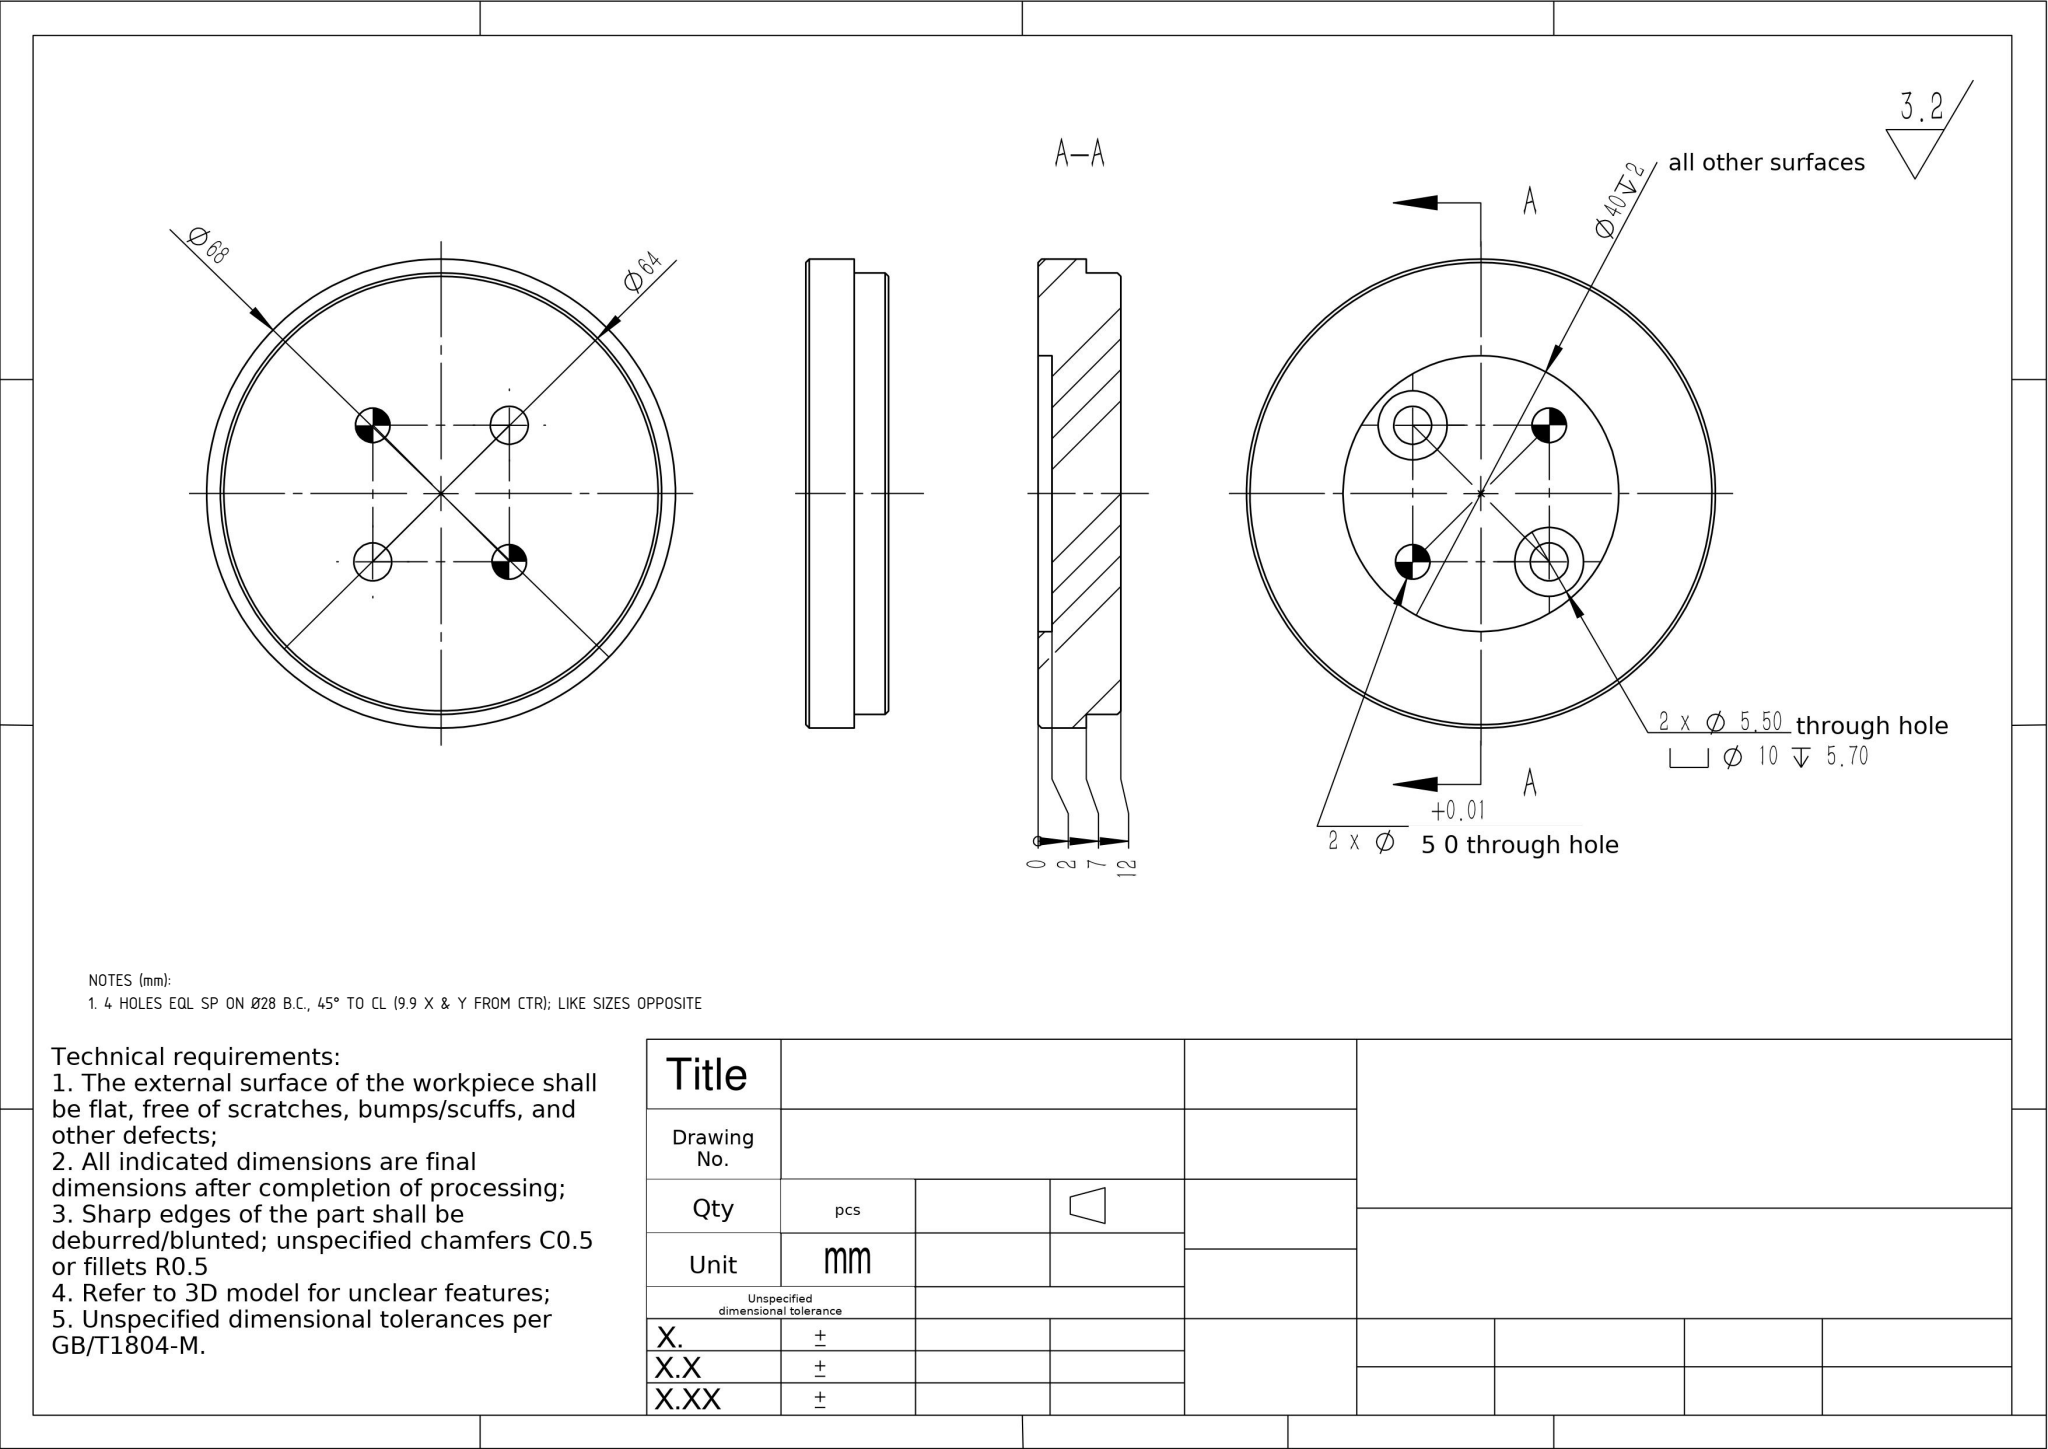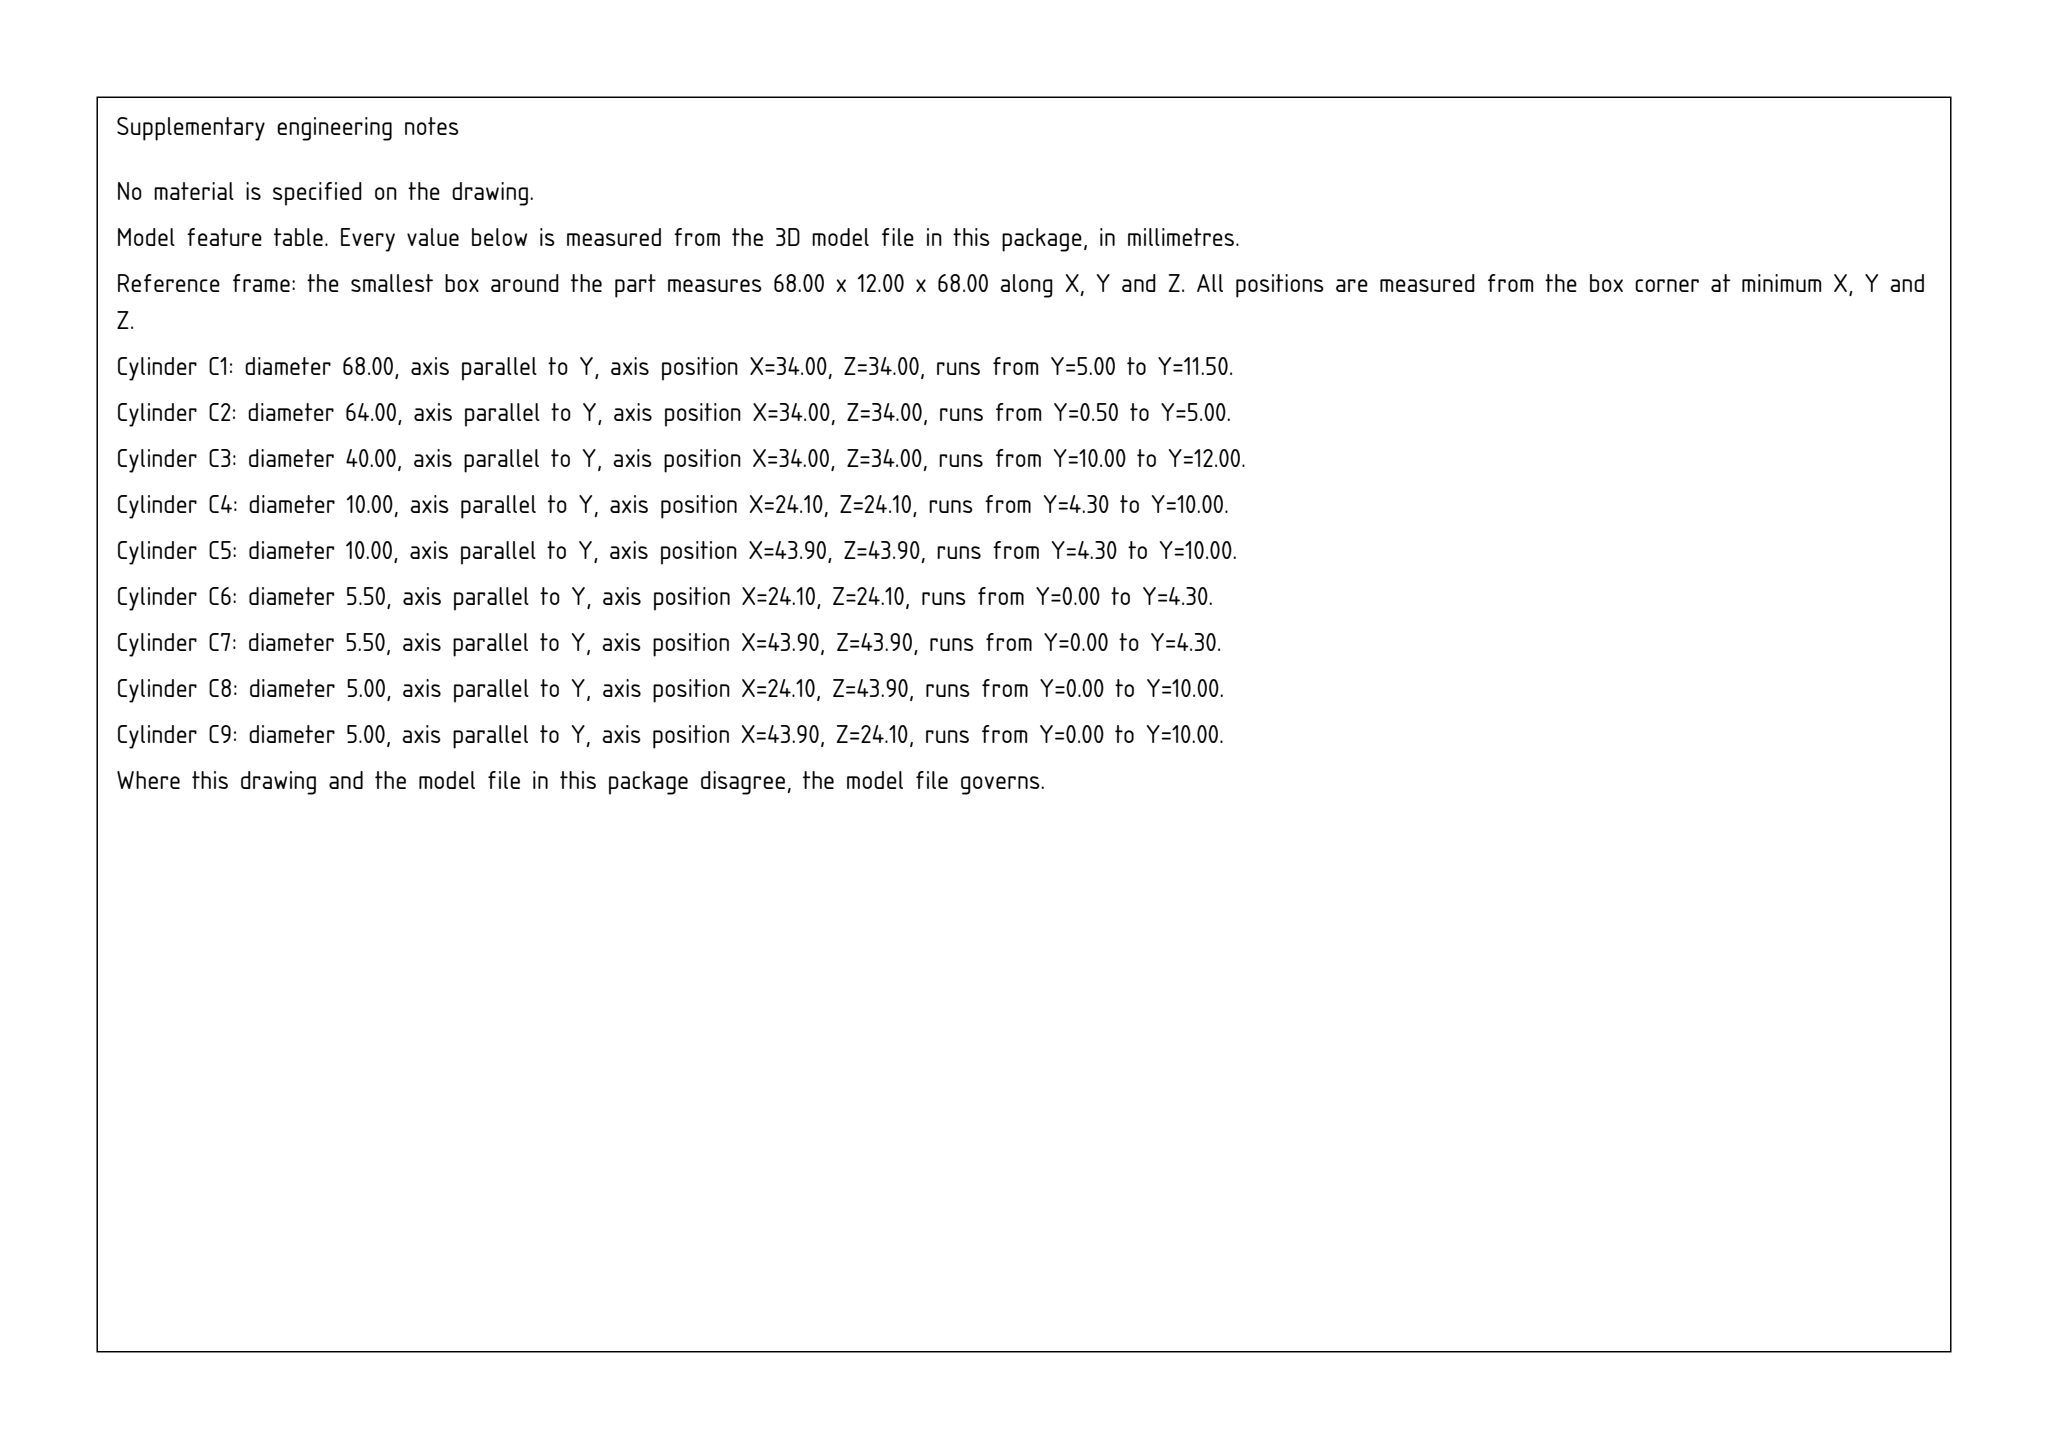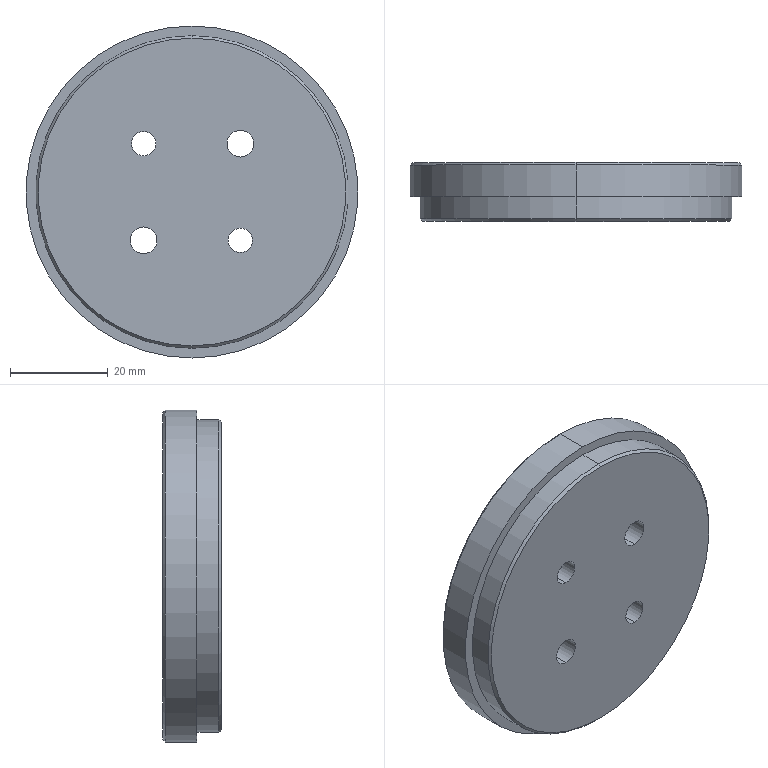Part | SolidWorks | mm | 1 solid | 28 faces | box 68 x 12 x 68 mm | volume 37449 mm3 | cylinder 18 | plane 6 | cone 4 | commonest cylinder face diameters 5 x4 10 x4 5.5 x4 40 x2 64 x2 68 x2
Drawing notes:
4 HOLES EQL SP ON Ø28 B.C., 45° TO CL (9.9 X & Y FROM CTR); LIKE SIZES OPPOSITE | from the solid: Ø5.5 at (24.1,24.1)&(43.9,43.9); Ø5.0 at (24.1,43.9)&(43.9,24.1); ctr 34,34; B.C.=2*sqrt(9.9²+9.9²)=28.0
build123d program:
from build123d import *

# Parameters (mm, degrees)
SKETCH1_R                                         = 34
BOSS_EXTRUDE1_DEPTH                               = 12
SKETCH5_R                                         = 34
SKETCH5_R_2                                       = 32
CUT_EXTRUDE2_DEPTH                                = 5
SKETCH9_R                                         = 20
CUT_EXTRUDE3_DEPTH                                = 2
HOLE_SIZE_ACCORDING_TO_HEXAGON_SOCKET_D           = 5.5
HOLE_SIZE_ACCORDING_TO_HEXAGON_SOCKET_CBORE_D     = 10
HOLE_SIZE_ACCORDING_TO_HEXAGON_SOCKET_CBORE_DEPTH = 5.7
SIZE_MM_DOWEL_PIN_HOLE_2_D                        = 5
CHAMFER1_SIZE                                     = 0.5


with BuildPart() as part:
    # Sketch1 → Boss-Extrude1 (new body)
    with BuildSketch(Plane(origin=(0, 0, 0), x_dir=(1, 0, 0), z_dir=(0, 1, 0))):
        with Locations(Location((0, 0, 0), (0, 0, 270))):
            Circle(SKETCH1_R)
    extrude(amount=BOSS_EXTRUDE1_DEPTH)

    # Sketch5 → Cut-Extrude2 (cut)
    with BuildSketch(Plane.XZ):
        with Locations(Location((0, 0, 0), (0, 0, 270))):
            Circle(SKETCH5_R)
        with Locations(Location((0, 0, 0), (0, 0, 270))):
            Circle(SKETCH5_R_2, mode=Mode.SUBTRACT)
    extrude(amount=-CUT_EXTRUDE2_DEPTH, mode=Mode.SUBTRACT)

    # Sketch9 → Cut-Extrude3 (cut)
    with BuildSketch(Plane(origin=(0, 12, 0), x_dir=(1, 0, 0), z_dir=(0, 1, 0))):
        with Locations(Location((0, 0, 0), (0, 0, 270))):
            Circle(SKETCH9_R)
    extrude(amount=-CUT_EXTRUDE3_DEPTH, mode=Mode.SUBTRACT)

    # Hole Size _ according to_ Hexagon Socket (through all)
    with Locations(Plane(origin=(-9.899, 10, -9.899), x_dir=(0, 0, 1), z_dir=(0, 1, 0))):
        with Locations((0, 0), (19.799, 19.799)):
            CounterBoreHole(HOLE_SIZE_ACCORDING_TO_HEXAGON_SOCKET_D / 2, HOLE_SIZE_ACCORDING_TO_HEXAGON_SOCKET_CBORE_D / 2, HOLE_SIZE_ACCORDING_TO_HEXAGON_SOCKET_CBORE_DEPTH)

    # Size mm Dowel Pin Hole 2 (through all)
    with Locations(Plane(origin=(-9.899, 10, 9.899), x_dir=(0, 0, 1), z_dir=(0, 1, 0))):
        with Locations((0, 0), (-19.799, 19.799)):
            Hole(SIZE_MM_DOWEL_PIN_HOLE_2_D / 2)

    # Chamfer1
    chamfer1_edges = [part.edges().sort_by_distance(p)[0] for p in [
        (0, 12, -34),
        (0, 0, 32),
    ]]
    chamfer(chamfer1_edges, length=CHAMFER1_SIZE)


solid = part.part
STEP:
#1=CARTESIAN_POINT('',(0.,12.,33.5));
#2=VERTEX_POINT('',#1);
#3=CARTESIAN_POINT('',(0.,12.,-33.5));
#4=VERTEX_POINT('',#3);
#5=CARTESIAN_POINT('',(0.,12.,0.));
#6=DIRECTION('',(0.,1.,0.));
#7=DIRECTION('',(0.,0.,1.));
#8=AXIS2_PLACEMENT_3D('',#5,#6,#7);
#9=CIRCLE('',#8,33.5);
#10=EDGE_CURVE('',#2,#4,#9,.T.);
#11=ORIENTED_EDGE('',*,*,#10,.F.);
#12=CARTESIAN_POINT('',(0.,11.5,34.));
#13=VERTEX_POINT('',#12);
#14=CARTESIAN_POINT('',(0.,12.,33.5));
#15=DIRECTION('',(0.,-0.7071,0.7071));
#16=VECTOR('',#15,1000.);
#17=LINE('',#14,#16);
#18=EDGE_CURVE('',#2,#13,#17,.T.);
#19=ORIENTED_EDGE('',*,*,#18,.T.);
#20=CARTESIAN_POINT('',(0.,11.5,-34.));
#21=VERTEX_POINT('',#20);
#22=CARTESIAN_POINT('',(0.,11.5,0.));
#23=DIRECTION('',(0.,-1.,0.));
#24=DIRECTION('',(0.,0.,1.));
#25=AXIS2_PLACEMENT_3D('',#22,#23,#24);
#26=CIRCLE('',#25,34.);
#27=EDGE_CURVE('',#21,#13,#26,.T.);
#28=ORIENTED_EDGE('',*,*,#27,.F.);
#29=CARTESIAN_POINT('',(0.,12.,-33.5));
#30=DIRECTION('',(0.,-0.7071,-0.7071));
#31=VECTOR('',#30,1000.);
#32=LINE('',#29,#31);
#33=EDGE_CURVE('',#4,#21,#32,.T.);
#34=ORIENTED_EDGE('',*,*,#33,.F.);
#35=EDGE_LOOP('',(#11,#19,#28,#34));
#36=FACE_OUTER_BOUND('',#35,.T.);
#37=CARTESIAN_POINT('',(0.,12.,0.));
#38=DIRECTION('',(0.,-1.,0.));
#39=DIRECTION('',(0.,0.,-1.));
#40=AXIS2_PLACEMENT_3D('',#37,#38,#39);
#41=CONICAL_SURFACE('',#40,33.5,0.7854);
#42=ADVANCED_FACE('',(#36),#41,.T.);
#43=CARTESIAN_POINT('',(0.,0.,-31.5));
#44=VERTEX_POINT('',#43);
#45=CARTESIAN_POINT('',(0.,0.,31.5));
#46=VERTEX_POINT('',#45);
#47=CARTESIAN_POINT('',(0.,0.,0.));
#48=DIRECTION('',(0.,-1.,0.));
#49=DIRECTION('',(0.,0.,1.));
#50=AXIS2_PLACEMENT_3D('',#47,#48,#49);
#51=CIRCLE('',#50,31.5);
#52=EDGE_CURVE('',#44,#46,#51,.T.);
#53=ORIENTED_EDGE('',*,*,#52,.F.);
#54=CARTESIAN_POINT('',(0.,0.5,-32.));
#55=VERTEX_POINT('',#54);
#56=CARTESIAN_POINT('',(0.,0.,-31.5));
#57=DIRECTION('',(0.,0.7071,-0.7071));
#58=VECTOR('',#57,1000.);
#59=LINE('',#56,#58);
#60=EDGE_CURVE('',#44,#55,#59,.T.);
#61=ORIENTED_EDGE('',*,*,#60,.T.);
#62=CARTESIAN_POINT('',(0.,0.5,32.));
#63=VERTEX_POINT('',#62);
#64=CARTESIAN_POINT('',(0.,0.5,0.));
#65=DIRECTION('',(0.,1.,0.));
#66=DIRECTION('',(0.,0.,1.));
#67=AXIS2_PLACEMENT_3D('',#64,#65,#66);
#68=CIRCLE('',#67,32.);
#69=EDGE_CURVE('',#63,#55,#68,.T.);
#70=ORIENTED_EDGE('',*,*,#69,.F.);
#71=CARTESIAN_POINT('',(0.,0.,31.5));
#72=DIRECTION('',(0.,0.7071,0.7071));
#73=VECTOR('',#72,1000.);
#74=LINE('',#71,#73);
#75=EDGE_CURVE('',#46,#63,#74,.T.);
#76=ORIENTED_EDGE('',*,*,#75,.F.);
#77=EDGE_LOOP('',(#53,#61,#70,#76));
#78=FACE_OUTER_BOUND('',#77,.T.);
#79=CARTESIAN_POINT('',(0.,0.,0.));
#80=DIRECTION('',(0.,1.,0.));
#81=DIRECTION('',(0.,0.,1.));
#82=AXIS2_PLACEMENT_3D('',#79,#80,#81);
#83=CONICAL_SURFACE('',#82,31.5,0.7854);
#84=ADVANCED_FACE('',(#78),#83,.T.);
#85=CARTESIAN_POINT('',(-9.899,0.,7.399));
#86=VERTEX_POINT('',#85);
#87=CARTESIAN_POINT('',(-9.899,0.,12.399));
#88=VERTEX_POINT('',#87);
#89=CARTESIAN_POINT('',(-9.899,0.,9.899));
#90=DIRECTION('',(0.,1.,0.));
#91=DIRECTION('',(0.,0.,1.));
#92=AXIS2_PLACEMENT_3D('',#89,#90,#91);
#93=CIRCLE('',#92,2.5);
#94=EDGE_CURVE('',#86,#88,#93,.T.);
#95=ORIENTED_EDGE('',*,*,#94,.F.);
#96=CARTESIAN_POINT('',(-9.899,10.,7.399));
#97=VERTEX_POINT('',#96);
#98=CARTESIAN_POINT('',(-9.899,10.,7.399));
#99=DIRECTION('',(0.,1.,0.));
#100=VECTOR('',#99,1000.);
#101=LINE('',#98,#100);
#102=EDGE_CURVE('',#86,#97,#101,.T.);
#103=ORIENTED_EDGE('',*,*,#102,.T.);
#104=CARTESIAN_POINT('',(-9.899,10.,12.399));
#105=VERTEX_POINT('',#104);
#106=CARTESIAN_POINT('',(-9.899,10.,9.899));
#107=DIRECTION('',(0.,1.,0.));
#108=DIRECTION('',(0.,0.,1.));
#109=AXIS2_PLACEMENT_3D('',#106,#107,#108);
#110=CIRCLE('',#109,2.5);
#111=EDGE_CURVE('',#97,#105,#110,.T.);
#112=ORIENTED_EDGE('',*,*,#111,.T.);
#113=CARTESIAN_POINT('',(-9.899,10.,12.399));
#114=DIRECTION('',(0.,1.,0.));
#115=VECTOR('',#114,1000.);
#116=LINE('',#113,#115);
#117=EDGE_CURVE('',#88,#105,#116,.T.);
#118=ORIENTED_EDGE('',*,*,#117,.F.);
#119=EDGE_LOOP('',(#95,#103,#112,#118));
#120=FACE_OUTER_BOUND('',#119,.T.);
#121=CARTESIAN_POINT('',(-9.899,10.,9.899));
#122=DIRECTION('',(0.,1.,0.));
#123=DIRECTION('',(0.,0.,1.));
#124=AXIS2_PLACEMENT_3D('',#121,#122,#123);
#125=CYLINDRICAL_SURFACE('',#124,2.5);
#126=ADVANCED_FACE('',(#120),#125,.F.);
#127=CARTESIAN_POINT('',(9.899,0.,-12.399));
#128=VERTEX_POINT('',#127);
#129=CARTESIAN_POINT('',(9.899,0.,-7.399));
#130=VERTEX_POINT('',#129);
#131=CARTESIAN_POINT('',(9.899,0.,-9.899));
#132=DIRECTION('',(0.,1.,0.));
#133=DIRECTION('',(0.,0.,1.));
#134=AXIS2_PLACEMENT_3D('',#131,#132,#133);
#135=CIRCLE('',#134,2.5);
#136=EDGE_CURVE('',#128,#130,#135,.T.);
#137=ORIENTED_EDGE('',*,*,#136,.F.);
#138=CARTESIAN_POINT('',(9.899,10.,-12.399));
#139=VERTEX_POINT('',#138);
#140=CARTESIAN_POINT('',(9.899,10.,-12.399));
#141=DIRECTION('',(0.,1.,0.));
#142=VECTOR('',#141,1000.);
#143=LINE('',#140,#142);
#144=EDGE_CURVE('',#128,#139,#143,.T.);
#145=ORIENTED_EDGE('',*,*,#144,.T.);
#146=CARTESIAN_POINT('',(9.899,10.,-7.399));
#147=VERTEX_POINT('',#146);
#148=CARTESIAN_POINT('',(9.899,10.,-9.899));
#149=DIRECTION('',(0.,1.,0.));
#150=DIRECTION('',(0.,0.,1.));
#151=AXIS2_PLACEMENT_3D('',#148,#149,#150);
#152=CIRCLE('',#151,2.5);
#153=EDGE_CURVE('',#139,#147,#152,.T.);
#154=ORIENTED_EDGE('',*,*,#153,.T.);
#155=CARTESIAN_POINT('',(9.899,10.,-7.399));
#156=DIRECTION('',(0.,1.,0.));
#157=VECTOR('',#156,1000.);
#158=LINE('',#155,#157);
#159=EDGE_CURVE('',#130,#147,#158,.T.);
#160=ORIENTED_EDGE('',*,*,#159,.F.);
#161=EDGE_LOOP('',(#137,#145,#154,#160));
#162=FACE_OUTER_BOUND('',#161,.T.);
#163=CARTESIAN_POINT('',(9.899,10.,-9.899));
#164=DIRECTION('',(0.,1.,0.));
#165=DIRECTION('',(0.,0.,1.));
#166=AXIS2_PLACEMENT_3D('',#163,#164,#165);
#167=CYLINDRICAL_SURFACE('',#166,2.5);
#168=ADVANCED_FACE('',(#162),#167,.F.);
#169=CARTESIAN_POINT('',(-9.899,4.3,-14.899));
#170=VERTEX_POINT('',#169);
#171=CARTESIAN_POINT('',(-9.899,4.3,-4.899));
#172=VERTEX_POINT('',#171);
#173=CARTESIAN_POINT('',(-9.899,4.3,-9.899));
#174=DIRECTION('',(0.,1.,0.));
#175=DIRECTION('',(0.,0.,1.));
#176=AXIS2_PLACEMENT_3D('',#173,#174,#175);
#177=CIRCLE('',#176,5.);
#178=EDGE_CURVE('',#170,#172,#177,.T.);
#179=ORIENTED_EDGE('',*,*,#178,.F.);
#180=CARTESIAN_POINT('',(-9.899,10.,-14.899));
#181=VERTEX_POINT('',#180);
#182=CARTESIAN_POINT('',(-9.899,10.,-14.899));
#183=DIRECTION('',(0.,1.,0.));
#184=VECTOR('',#183,1000.);
#185=LINE('',#182,#184);
#186=EDGE_CURVE('',#170,#181,#185,.T.);
#187=ORIENTED_EDGE('',*,*,#186,.T.);
#188=CARTESIAN_POINT('',(-9.899,10.,-4.899));
#189=VERTEX_POINT('',#188);
#190=CARTESIAN_POINT('',(-9.899,10.,-9.899));
#191=DIRECTION('',(0.,1.,0.));
#192=DIRECTION('',(0.,0.,1.));
#193=AXIS2_PLACEMENT_3D('',#190,#191,#192);
#194=CIRCLE('',#193,5.);
#195=EDGE_CURVE('',#181,#189,#194,.T.);
#196=ORIENTED_EDGE('',*,*,#195,.T.);
#197=CARTESIAN_POINT('',(-9.899,10.,-4.899));
#198=DIRECTION('',(0.,1.,0.));
#199=VECTOR('',#198,1000.);
#200=LINE('',#197,#199);
#201=EDGE_CURVE('',#172,#189,#200,.T.);
#202=ORIENTED_EDGE('',*,*,#201,.F.);
#203=EDGE_LOOP('',(#179,#187,#196,#202));
#204=FACE_OUTER_BOUND('',#203,.T.);
#205=CARTESIAN_POINT('',(-9.899,10.,-9.899));
#206=DIRECTION('',(0.,1.,0.));
#207=DIRECTION('',(0.,0.,1.));
#208=AXIS2_PLACEMENT_3D('',#205,#206,#207);
#209=CYLINDRICAL_SURFACE('',#208,5.);
#210=ADVANCED_FACE('',(#204),#209,.F.);
#211=CARTESIAN_POINT('',(-9.899,0.,-12.649));
#212=VERTEX_POINT('',#211);
#213=CARTESIAN_POINT('',(-9.899,0.,-7.149));
#214=VERTEX_POINT('',#213);
#215=CARTESIAN_POINT('',(-9.899,0.,-9.899));
#216=DIRECTION('',(0.,1.,0.));
#217=DIRECTION('',(0.,0.,1.));
#218=AXIS2_PLACEMENT_3D('',#215,#216,#217);
#219=CIRCLE('',#218,2.75);
#220=EDGE_CURVE('',#212,#214,#219,.T.);
#221=ORIENTED_EDGE('',*,*,#220,.F.);
#222=CARTESIAN_POINT('',(-9.899,4.3,-12.649));
#223=VERTEX_POINT('',#222);
#224=CARTESIAN_POINT('',(-9.899,10.,-12.649));
#225=DIRECTION('',(0.,1.,0.));
#226=VECTOR('',#225,1000.);
#227=LINE('',#224,#226);
#228=EDGE_CURVE('',#212,#223,#227,.T.);
#229=ORIENTED_EDGE('',*,*,#228,.T.);
#230=CARTESIAN_POINT('',(-9.899,4.3,-7.149));
#231=VERTEX_POINT('',#230);
#232=CARTESIAN_POINT('',(-9.899,4.3,-9.899));
#233=DIRECTION('',(0.,1.,0.));
#234=DIRECTION('',(0.,0.,1.));
#235=AXIS2_PLACEMENT_3D('',#232,#233,#234);
#236=CIRCLE('',#235,2.75);
#237=EDGE_CURVE('',#223,#231,#236,.T.);
#238=ORIENTED_EDGE('',*,*,#237,.T.);
#239=CARTESIAN_POINT('',(-9.899,10.,-7.149));
#240=DIRECTION('',(0.,1.,0.));
#241=VECTOR('',#240,1000.);
#242=LINE('',#239,#241);
#243=EDGE_CURVE('',#214,#231,#242,.T.);
#244=ORIENTED_EDGE('',*,*,#243,.F.);
#245=EDGE_LOOP('',(#221,#229,#238,#244));
#246=FACE_OUTER_BOUND('',#245,.T.);
#247=CARTESIAN_POINT('',(-9.899,10.,-9.899));
#248=DIRECTION('',(0.,1.,0.));
#249=DIRECTION('',(0.,0.,1.));
#250=AXIS2_PLACEMENT_3D('',#247,#248,#249);
#251=CYLINDRICAL_SURFACE('',#250,2.75);
#252=ADVANCED_FACE('',(#246),#251,.F.);
#253=CARTESIAN_POINT('',(9.899,4.3,4.899));
#254=VERTEX_POINT('',#253);
#255=CARTESIAN_POINT('',(9.899,4.3,14.899));
#256=VERTEX_POINT('',#255);
#257=CARTESIAN_POINT('',(9.899,4.3,9.899));
#258=DIRECTION('',(0.,1.,0.));
#259=DIRECTION('',(0.,0.,1.));
#260=AXIS2_PLACEMENT_3D('',#257,#258,#259);
#261=CIRCLE('',#260,5.);
#262=EDGE_CURVE('',#254,#256,#261,.T.);
#263=ORIENTED_EDGE('',*,*,#262,.F.);
#264=CARTESIAN_POINT('',(9.899,10.,4.899));
#265=VERTEX_POINT('',#264);
#266=CARTESIAN_POINT('',(9.899,10.,4.899));
#267=DIRECTION('',(0.,1.,0.));
#268=VECTOR('',#267,1000.);
#269=LINE('',#266,#268);
#270=EDGE_CURVE('',#254,#265,#269,.T.);
#271=ORIENTED_EDGE('',*,*,#270,.T.);
#272=CARTESIAN_POINT('',(9.899,10.,14.899));
#273=VERTEX_POINT('',#272);
#274=CARTESIAN_POINT('',(9.899,10.,9.899));
#275=DIRECTION('',(0.,1.,0.));
#276=DIRECTION('',(0.,0.,1.));
#277=AXIS2_PLACEMENT_3D('',#274,#275,#276);
#278=CIRCLE('',#277,5.);
#279=EDGE_CURVE('',#265,#273,#278,.T.);
#280=ORIENTED_EDGE('',*,*,#279,.T.);
#281=CARTESIAN_POINT('',(9.899,10.,14.899));
#282=DIRECTION('',(0.,1.,0.));
#283=VECTOR('',#282,1000.);
#284=LINE('',#281,#283);
#285=EDGE_CURVE('',#256,#273,#284,.T.);
#286=ORIENTED_EDGE('',*,*,#285,.F.);
#287=EDGE_LOOP('',(#263,#271,#280,#286));
#288=FACE_OUTER_BOUND('',#287,.T.);
#289=CARTESIAN_POINT('',(9.899,10.,9.899));
#290=DIRECTION('',(0.,1.,0.));
#291=DIRECTION('',(0.,0.,1.));
#292=AXIS2_PLACEMENT_3D('',#289,#290,#291);
#293=CYLINDRICAL_SURFACE('',#292,5.);
#294=ADVANCED_FACE('',(#288),#293,.F.);
#295=CARTESIAN_POINT('',(9.899,0.,7.149));
#296=VERTEX_POINT('',#295);
#297=CARTESIAN_POINT('',(9.899,0.,12.649));
#298=VERTEX_POINT('',#297);
#299=CARTESIAN_POINT('',(9.899,0.,9.899));
#300=DIRECTION('',(0.,1.,0.));
#301=DIRECTION('',(0.,0.,1.));
#302=AXIS2_PLACEMENT_3D('',#299,#300,#301);
#303=CIRCLE('',#302,2.75);
#304=EDGE_CURVE('',#296,#298,#303,.T.);
#305=ORIENTED_EDGE('',*,*,#304,.F.);
#306=CARTESIAN_POINT('',(9.899,4.3,7.149));
#307=VERTEX_POINT('',#306);
#308=CARTESIAN_POINT('',(9.899,10.,7.149));
#309=DIRECTION('',(0.,1.,0.));
#310=VECTOR('',#309,1000.);
#311=LINE('',#308,#310);
#312=EDGE_CURVE('',#296,#307,#311,.T.);
#313=ORIENTED_EDGE('',*,*,#312,.T.);
#314=CARTESIAN_POINT('',(9.899,4.3,12.649));
#315=VERTEX_POINT('',#314);
#316=CARTESIAN_POINT('',(9.899,4.3,9.899));
#317=DIRECTION('',(0.,1.,0.));
#318=DIRECTION('',(0.,0.,1.));
#319=AXIS2_PLACEMENT_3D('',#316,#317,#318);
#320=CIRCLE('',#319,2.75);
#321=EDGE_CURVE('',#307,#315,#320,.T.);
#322=ORIENTED_EDGE('',*,*,#321,.T.);
#323=CARTESIAN_POINT('',(9.899,10.,12.649));
#324=DIRECTION('',(0.,1.,0.));
#325=VECTOR('',#324,1000.);
#326=LINE('',#323,#325);
#327=EDGE_CURVE('',#298,#315,#326,.T.);
#328=ORIENTED_EDGE('',*,*,#327,.F.);
#329=EDGE_LOOP('',(#305,#313,#322,#328));
#330=FACE_OUTER_BOUND('',#329,.T.);
#331=CARTESIAN_POINT('',(9.899,10.,9.899));
#332=DIRECTION('',(0.,1.,0.));
#333=DIRECTION('',(0.,0.,1.));
#334=AXIS2_PLACEMENT_3D('',#331,#332,#333);
#335=CYLINDRICAL_SURFACE('',#334,2.75);
#336=ADVANCED_FACE('',(#330),#335,.F.);
#337=CARTESIAN_POINT('',(0.,10.,-20.));
#338=VERTEX_POINT('',#337);
#339=CARTESIAN_POINT('',(0.,10.,20.));
#340=VERTEX_POINT('',#339);
#341=CARTESIAN_POINT('',(0.,10.,0.));
#342=DIRECTION('',(0.,1.,0.));
#343=DIRECTION('',(0.,0.,1.));
#344=AXIS2_PLACEMENT_3D('',#341,#342,#343);
#345=CIRCLE('',#344,20.);
#346=EDGE_CURVE('',#338,#340,#345,.T.);
#347=ORIENTED_EDGE('',*,*,#346,.F.);
#348=CARTESIAN_POINT('',(0.,12.,-20.));
#349=VERTEX_POINT('',#348);
#350=CARTESIAN_POINT('',(0.,10.,-20.));
#351=DIRECTION('',(0.,1.,0.));
#352=VECTOR('',#351,1000.);
#353=LINE('',#350,#352);
#354=EDGE_CURVE('',#338,#349,#353,.T.);
#355=ORIENTED_EDGE('',*,*,#354,.T.);
#356=CARTESIAN_POINT('',(0.,12.,20.));
#357=VERTEX_POINT('',#356);
#358=CARTESIAN_POINT('',(0.,12.,0.));
#359=DIRECTION('',(0.,1.,0.));
#360=DIRECTION('',(0.,0.,1.));
#361=AXIS2_PLACEMENT_3D('',#358,#359,#360);
#362=CIRCLE('',#361,20.);
#363=EDGE_CURVE('',#349,#357,#362,.T.);
#364=ORIENTED_EDGE('',*,*,#363,.T.);
#365=CARTESIAN_POINT('',(0.,10.,20.));
#366=DIRECTION('',(0.,1.,0.));
#367=VECTOR('',#366,1000.);
#368=LINE('',#365,#367);
#369=EDGE_CURVE('',#340,#357,#368,.T.);
#370=ORIENTED_EDGE('',*,*,#369,.F.);
#371=EDGE_LOOP('',(#347,#355,#364,#370));
#372=FACE_OUTER_BOUND('',#371,.T.);
#373=CARTESIAN_POINT('',(0.,10.,0.));
#374=DIRECTION('',(0.,1.,0.));
#375=DIRECTION('',(0.,0.,1.));
#376=AXIS2_PLACEMENT_3D('',#373,#374,#375);
#377=CYLINDRICAL_SURFACE('',#376,20.);
#378=ADVANCED_FACE('',(#372),#377,.F.);
#379=CARTESIAN_POINT('',(0.,5.,-32.));
#380=VERTEX_POINT('',#379);
#381=CARTESIAN_POINT('',(0.,5.,32.));
#382=VERTEX_POINT('',#381);
#383=CARTESIAN_POINT('',(0.,5.,0.));
#384=DIRECTION('',(0.,-1.,0.));
#385=DIRECTION('',(0.,0.,-1.));
#386=AXIS2_PLACEMENT_3D('',#383,#384,#385);
#387=CIRCLE('',#386,32.);
#388=EDGE_CURVE('',#380,#382,#387,.T.);
#389=ORIENTED_EDGE('',*,*,#388,.T.);
#390=CARTESIAN_POINT('',(0.,5.,32.));
#391=DIRECTION('',(0.,-1.,0.));
#392=VECTOR('',#391,1000.);
#393=LINE('',#390,#392);
#394=EDGE_CURVE('',#382,#63,#393,.T.);
#395=ORIENTED_EDGE('',*,*,#394,.T.);
#396=ORIENTED_EDGE('',*,*,#69,.T.);
#397=CARTESIAN_POINT('',(0.,5.,-32.));
#398=DIRECTION('',(0.,-1.,0.));
#399=VECTOR('',#398,1000.);
#400=LINE('',#397,#399);
#401=EDGE_CURVE('',#380,#55,#400,.T.);
#402=ORIENTED_EDGE('',*,*,#401,.F.);
#403=EDGE_LOOP('',(#389,#395,#396,#402));
#404=FACE_OUTER_BOUND('',#403,.T.);
#405=CARTESIAN_POINT('',(0.,5.,0.));
#406=DIRECTION('',(0.,-1.,0.));
#407=DIRECTION('',(0.,0.,-1.));
#408=AXIS2_PLACEMENT_3D('',#405,#406,#407);
#409=CYLINDRICAL_SURFACE('',#408,32.);
#410=ADVANCED_FACE('',(#404),#409,.T.);
#411=ORIENTED_EDGE('',*,*,#27,.T.);
#412=CARTESIAN_POINT('',(0.,5.,34.));
#413=VERTEX_POINT('',#412);
#414=CARTESIAN_POINT('',(0.,12.,34.));
#415=DIRECTION('',(0.,-1.,0.));
#416=VECTOR('',#415,1000.);
#417=LINE('',#414,#416);
#418=EDGE_CURVE('',#13,#413,#417,.T.);
#419=ORIENTED_EDGE('',*,*,#418,.T.);
#420=CARTESIAN_POINT('',(0.,5.,-34.));
#421=VERTEX_POINT('',#420);
#422=CARTESIAN_POINT('',(0.,5.,0.));
#423=DIRECTION('',(0.,-1.,0.));
#424=DIRECTION('',(0.,0.,-1.));
#425=AXIS2_PLACEMENT_3D('',#422,#423,#424);
#426=CIRCLE('',#425,34.);
#427=EDGE_CURVE('',#421,#413,#426,.T.);
#428=ORIENTED_EDGE('',*,*,#427,.F.);
#429=CARTESIAN_POINT('',(0.,12.,-34.));
#430=DIRECTION('',(0.,-1.,0.));
#431=VECTOR('',#430,1000.);
#432=LINE('',#429,#431);
#433=EDGE_CURVE('',#21,#421,#432,.T.);
#434=ORIENTED_EDGE('',*,*,#433,.F.);
#435=EDGE_LOOP('',(#411,#419,#428,#434));
#436=FACE_OUTER_BOUND('',#435,.T.);
#437=CARTESIAN_POINT('',(0.,12.,0.));
#438=DIRECTION('',(0.,-1.,0.));
#439=DIRECTION('',(0.,0.,-1.));
#440=AXIS2_PLACEMENT_3D('',#437,#438,#439);
#441=CYLINDRICAL_SURFACE('',#440,34.);
#442=ADVANCED_FACE('',(#436),#441,.T.);
#443=ORIENTED_EDGE('',*,*,#418,.F.);
#444=CARTESIAN_POINT('',(0.,11.5,0.));
#445=DIRECTION('',(0.,-1.,0.));
#446=DIRECTION('',(0.,0.,1.));
#447=AXIS2_PLACEMENT_3D('',#444,#445,#446);
#448=CIRCLE('',#447,34.);
#449=EDGE_CURVE('',#13,#21,#448,.T.);
#450=ORIENTED_EDGE('',*,*,#449,.T.);
#451=ORIENTED_EDGE('',*,*,#433,.T.);
#452=CARTESIAN_POINT('',(0.,5.,0.));
#453=DIRECTION('',(0.,-1.,0.));
#454=DIRECTION('',(0.,0.,-1.));
#455=AXIS2_PLACEMENT_3D('',#452,#453,#454);
#456=CIRCLE('',#455,34.);
#457=EDGE_CURVE('',#413,#421,#456,.T.);
#458=ORIENTED_EDGE('',*,*,#457,.F.);
#459=EDGE_LOOP('',(#443,#450,#451,#458));
#460=FACE_OUTER_BOUND('',#459,.T.);
#461=CARTESIAN_POINT('',(0.,12.,0.));
#462=DIRECTION('',(0.,-1.,0.));
#463=DIRECTION('',(0.,0.,-1.));
#464=AXIS2_PLACEMENT_3D('',#461,#462,#463);
#465=CYLINDRICAL_SURFACE('',#464,34.);
#466=ADVANCED_FACE('',(#460),#465,.T.);
#467=CARTESIAN_POINT('',(0.,12.,0.));
#468=DIRECTION('',(0.,1.,0.));
#469=DIRECTION('',(0.,0.,1.));
#470=AXIS2_PLACEMENT_3D('',#467,#468,#469);
#471=CIRCLE('',#470,33.5);
#472=EDGE_CURVE('',#4,#2,#471,.T.);
#473=ORIENTED_EDGE('',*,*,#472,.T.);
#474=ORIENTED_EDGE('',*,*,#10,.T.);
#475=EDGE_LOOP('',(#473,#474));
#476=FACE_OUTER_BOUND('',#475,.T.);
#477=CARTESIAN_POINT('',(0.,12.,0.));
#478=DIRECTION('',(0.,1.,0.));
#479=DIRECTION('',(0.,0.,1.));
#480=AXIS2_PLACEMENT_3D('',#477,#478,#479);
#481=CIRCLE('',#480,20.);
#482=EDGE_CURVE('',#357,#349,#481,.T.);
#483=ORIENTED_EDGE('',*,*,#482,.F.);
#484=ORIENTED_EDGE('',*,*,#363,.F.);
#485=EDGE_LOOP('',(#483,#484));
#486=FACE_BOUND('',#485,.T.);
#487=CARTESIAN_POINT('',(0.,12.,0.));
#488=DIRECTION('',(0.,1.,0.));
#489=DIRECTION('',(0.,0.,1.));
#490=AXIS2_PLACEMENT_3D('',#487,#488,#489);
#491=PLANE('',#490);
#492=ADVANCED_FACE('',(#476,#486),#491,.T.);
#493=ORIENTED_EDGE('',*,*,#388,.F.);
#494=CARTESIAN_POINT('',(0.,5.,0.));
#495=DIRECTION('',(0.,-1.,0.));
#496=DIRECTION('',(0.,0.,-1.));
#497=AXIS2_PLACEMENT_3D('',#494,#495,#496);
#498=CIRCLE('',#497,32.);
#499=EDGE_CURVE('',#382,#380,#498,.T.);
#500=ORIENTED_EDGE('',*,*,#499,.F.);
#501=EDGE_LOOP('',(#493,#500));
#502=FACE_BOUND('',#501,.T.);
#503=ORIENTED_EDGE('',*,*,#427,.T.);
#504=ORIENTED_EDGE('',*,*,#457,.T.);
#505=EDGE_LOOP('',(#503,#504));
#506=FACE_OUTER_BOUND('',#505,.T.);
#507=CARTESIAN_POINT('',(0.,5.,0.));
#508=DIRECTION('',(0.,-1.,0.));
#509=DIRECTION('',(0.,0.,-1.));
#510=AXIS2_PLACEMENT_3D('',#507,#508,#509);
#511=PLANE('',#510);
#512=ADVANCED_FACE('',(#502,#506),#511,.T.);
#513=ORIENTED_EDGE('',*,*,#394,.F.);
#514=ORIENTED_EDGE('',*,*,#499,.T.);
#515=ORIENTED_EDGE('',*,*,#401,.T.);
#516=CARTESIAN_POINT('',(0.,0.5,0.));
#517=DIRECTION('',(0.,1.,0.));
#518=DIRECTION('',(0.,0.,1.));
#519=AXIS2_PLACEMENT_3D('',#516,#517,#518);
#520=CIRCLE('',#519,32.);
#521=EDGE_CURVE('',#55,#63,#520,.T.);
#522=ORIENTED_EDGE('',*,*,#521,.T.);
#523=EDGE_LOOP('',(#513,#514,#515,#522));
#524=FACE_OUTER_BOUND('',#523,.T.);
#525=CARTESIAN_POINT('',(0.,5.,0.));
#526=DIRECTION('',(0.,-1.,0.));
#527=DIRECTION('',(0.,0.,-1.));
#528=AXIS2_PLACEMENT_3D('',#525,#526,#527);
#529=CYLINDRICAL_SURFACE('',#528,32.);
#530=ADVANCED_FACE('',(#524),#529,.T.);
#531=CARTESIAN_POINT('',(0.,0.,0.));
#532=DIRECTION('',(0.,-1.,0.));
#533=DIRECTION('',(0.,0.,1.));
#534=AXIS2_PLACEMENT_3D('',#531,#532,#533);
#535=CIRCLE('',#534,31.5);
#536=EDGE_CURVE('',#46,#44,#535,.T.);
#537=ORIENTED_EDGE('',*,*,#536,.T.);
#538=ORIENTED_EDGE('',*,*,#52,.T.);
#539=EDGE_LOOP('',(#537,#538));
#540=FACE_OUTER_BOUND('',#539,.T.);
#541=CARTESIAN_POINT('',(-9.899,0.,9.899));
#542=DIRECTION('',(0.,1.,0.));
#543=DIRECTION('',(0.,0.,1.));
#544=AXIS2_PLACEMENT_3D('',#541,#542,#543);
#545=CIRCLE('',#544,2.5);
#546=EDGE_CURVE('',#88,#86,#545,.T.);
#547=ORIENTED_EDGE('',*,*,#546,.T.);
#548=ORIENTED_EDGE('',*,*,#94,.T.);
#549=EDGE_LOOP('',(#547,#548));
#550=FACE_BOUND('',#549,.T.);
#551=CARTESIAN_POINT('',(9.899,0.,-9.899));
#552=DIRECTION('',(0.,1.,0.));
#553=DIRECTION('',(0.,0.,1.));
#554=AXIS2_PLACEMENT_3D('',#551,#552,#553);
#555=CIRCLE('',#554,2.5);
#556=EDGE_CURVE('',#130,#128,#555,.T.);
#557=ORIENTED_EDGE('',*,*,#556,.T.);
#558=ORIENTED_EDGE('',*,*,#136,.T.);
#559=EDGE_LOOP('',(#557,#558));
#560=FACE_BOUND('',#559,.T.);
#561=CARTESIAN_POINT('',(-9.899,0.,-9.899));
#562=DIRECTION('',(0.,1.,0.));
#563=DIRECTION('',(0.,0.,1.));
#564=AXIS2_PLACEMENT_3D('',#561,#562,#563);
#565=CIRCLE('',#564,2.75);
#566=EDGE_CURVE('',#214,#212,#565,.T.);
#567=ORIENTED_EDGE('',*,*,#566,.T.);
#568=ORIENTED_EDGE('',*,*,#220,.T.);
#569=EDGE_LOOP('',(#567,#568));
#570=FACE_BOUND('',#569,.T.);
#571=CARTESIAN_POINT('',(9.899,0.,9.899));
#572=DIRECTION('',(0.,1.,0.));
#573=DIRECTION('',(0.,0.,1.));
#574=AXIS2_PLACEMENT_3D('',#571,#572,#573);
#575=CIRCLE('',#574,2.75);
#576=EDGE_CURVE('',#298,#296,#575,.T.);
#577=ORIENTED_EDGE('',*,*,#576,.T.);
#578=ORIENTED_EDGE('',*,*,#304,.T.);
#579=EDGE_LOOP('',(#577,#578));
#580=FACE_BOUND('',#579,.T.);
#581=CARTESIAN_POINT('',(0.,0.,0.));
#582=DIRECTION('',(0.,1.,0.));
#583=DIRECTION('',(0.,0.,1.));
#584=AXIS2_PLACEMENT_3D('',#581,#582,#583);
#585=PLANE('',#584);
#586=ADVANCED_FACE('',(#540,#550,#560,#570,#580),#585,.F.);
#587=ORIENTED_EDGE('',*,*,#354,.F.);
#588=CARTESIAN_POINT('',(0.,10.,0.));
#589=DIRECTION('',(0.,1.,0.));
#590=DIRECTION('',(0.,0.,1.));
#591=AXIS2_PLACEMENT_3D('',#588,#589,#590);
#592=CIRCLE('',#591,20.);
#593=EDGE_CURVE('',#340,#338,#592,.T.);
#594=ORIENTED_EDGE('',*,*,#593,.F.);
#595=ORIENTED_EDGE('',*,*,#369,.T.);
#596=ORIENTED_EDGE('',*,*,#482,.T.);
#597=EDGE_LOOP('',(#587,#594,#595,#596));
#598=FACE_OUTER_BOUND('',#597,.T.);
#599=CARTESIAN_POINT('',(0.,10.,0.));
#600=DIRECTION('',(0.,1.,0.));
#601=DIRECTION('',(0.,0.,1.));
#602=AXIS2_PLACEMENT_3D('',#599,#600,#601);
#603=CYLINDRICAL_SURFACE('',#602,20.);
#604=ADVANCED_FACE('',(#598),#603,.F.);
#605=CARTESIAN_POINT('',(-9.899,10.,9.899));
#606=DIRECTION('',(0.,1.,0.));
#607=DIRECTION('',(0.,0.,1.));
#608=AXIS2_PLACEMENT_3D('',#605,#606,#607);
#609=CIRCLE('',#608,2.5);
#610=EDGE_CURVE('',#105,#97,#609,.T.);
#611=ORIENTED_EDGE('',*,*,#610,.F.);
#612=ORIENTED_EDGE('',*,*,#111,.F.);
#613=EDGE_LOOP('',(#611,#612));
#614=FACE_BOUND('',#613,.T.);
#615=CARTESIAN_POINT('',(9.899,10.,-9.899));
#616=DIRECTION('',(0.,1.,0.));
#617=DIRECTION('',(0.,0.,1.));
#618=AXIS2_PLACEMENT_3D('',#615,#616,#617);
#619=CIRCLE('',#618,2.5);
#620=EDGE_CURVE('',#147,#139,#619,.T.);
#621=ORIENTED_EDGE('',*,*,#620,.F.);
#622=ORIENTED_EDGE('',*,*,#153,.F.);
#623=EDGE_LOOP('',(#621,#622));
#624=FACE_BOUND('',#623,.T.);
#625=CARTESIAN_POINT('',(-9.899,10.,-9.899));
#626=DIRECTION('',(0.,1.,0.));
#627=DIRECTION('',(0.,0.,1.));
#628=AXIS2_PLACEMENT_3D('',#625,#626,#627);
#629=CIRCLE('',#628,5.);
#630=EDGE_CURVE('',#189,#181,#629,.T.);
#631=ORIENTED_EDGE('',*,*,#630,.F.);
#632=ORIENTED_EDGE('',*,*,#195,.F.);
#633=EDGE_LOOP('',(#631,#632));
#634=FACE_BOUND('',#633,.T.);
#635=CARTESIAN_POINT('',(9.899,10.,9.899));
#636=DIRECTION('',(0.,1.,0.));
#637=DIRECTION('',(0.,0.,1.));
#638=AXIS2_PLACEMENT_3D('',#635,#636,#637);
#639=CIRCLE('',#638,5.);
#640=EDGE_CURVE('',#273,#265,#639,.T.);
#641=ORIENTED_EDGE('',*,*,#640,.F.);
#642=ORIENTED_EDGE('',*,*,#279,.F.);
#643=EDGE_LOOP('',(#641,#642));
#644=FACE_BOUND('',#643,.T.);
#645=ORIENTED_EDGE('',*,*,#593,.T.);
#646=ORIENTED_EDGE('',*,*,#346,.T.);
#647=EDGE_LOOP('',(#645,#646));
#648=FACE_OUTER_BOUND('',#647,.T.);
#649=CARTESIAN_POINT('',(0.,10.,0.));
#650=DIRECTION('',(0.,1.,0.));
#651=DIRECTION('',(0.,0.,1.));
#652=AXIS2_PLACEMENT_3D('',#649,#650,#651);
#653=PLANE('',#652);
#654=ADVANCED_FACE('',(#614,#624,#634,#644,#648),#653,.T.);
#655=ORIENTED_EDGE('',*,*,#312,.F.);
#656=ORIENTED_EDGE('',*,*,#576,.F.);
#657=ORIENTED_EDGE('',*,*,#327,.T.);
#658=CARTESIAN_POINT('',(9.899,4.3,9.899));
#659=DIRECTION('',(0.,1.,0.));
#660=DIRECTION('',(0.,0.,1.));
#661=AXIS2_PLACEMENT_3D('',#658,#659,#660);
#662=CIRCLE('',#661,2.75);
#663=EDGE_CURVE('',#315,#307,#662,.T.);
#664=ORIENTED_EDGE('',*,*,#663,.T.);
#665=EDGE_LOOP('',(#655,#656,#657,#664));
#666=FACE_OUTER_BOUND('',#665,.T.);
#667=CARTESIAN_POINT('',(9.899,10.,9.899));
#668=DIRECTION('',(0.,1.,0.));
#669=DIRECTION('',(0.,0.,1.));
#670=AXIS2_PLACEMENT_3D('',#667,#668,#669);
#671=CYLINDRICAL_SURFACE('',#670,2.75);
#672=ADVANCED_FACE('',(#666),#671,.F.);
#673=ORIENTED_EDGE('',*,*,#663,.F.);
#674=ORIENTED_EDGE('',*,*,#321,.F.);
#675=EDGE_LOOP('',(#673,#674));
#676=FACE_BOUND('',#675,.T.);
#677=CARTESIAN_POINT('',(9.899,4.3,9.899));
#678=DIRECTION('',(0.,1.,0.));
#679=DIRECTION('',(0.,0.,1.));
#680=AXIS2_PLACEMENT_3D('',#677,#678,#679);
#681=CIRCLE('',#680,5.);
#682=EDGE_CURVE('',#256,#254,#681,.T.);
#683=ORIENTED_EDGE('',*,*,#682,.T.);
#684=ORIENTED_EDGE('',*,*,#262,.T.);
#685=EDGE_LOOP('',(#683,#684));
#686=FACE_OUTER_BOUND('',#685,.T.);
#687=CARTESIAN_POINT('',(12.649,4.3,9.899));
#688=DIRECTION('',(0.,-1.,0.));
#689=DIRECTION('',(0.,0.,-1.));
#690=AXIS2_PLACEMENT_3D('',#687,#688,#689);
#691=PLANE('',#690);
#692=ADVANCED_FACE('',(#676,#686),#691,.F.);
#693=ORIENTED_EDGE('',*,*,#270,.F.);
#694=ORIENTED_EDGE('',*,*,#682,.F.);
#695=ORIENTED_EDGE('',*,*,#285,.T.);
#696=ORIENTED_EDGE('',*,*,#640,.T.);
#697=EDGE_LOOP('',(#693,#694,#695,#696));
#698=FACE_OUTER_BOUND('',#697,.T.);
#699=CARTESIAN_POINT('',(9.899,10.,9.899));
#700=DIRECTION('',(0.,1.,0.));
#701=DIRECTION('',(0.,0.,1.));
#702=AXIS2_PLACEMENT_3D('',#699,#700,#701);
#703=CYLINDRICAL_SURFACE('',#702,5.);
#704=ADVANCED_FACE('',(#698),#703,.F.);
#705=ORIENTED_EDGE('',*,*,#228,.F.);
#706=ORIENTED_EDGE('',*,*,#566,.F.);
#707=ORIENTED_EDGE('',*,*,#243,.T.);
#708=CARTESIAN_POINT('',(-9.899,4.3,-9.899));
#709=DIRECTION('',(0.,1.,0.));
#710=DIRECTION('',(0.,0.,1.));
#711=AXIS2_PLACEMENT_3D('',#708,#709,#710);
#712=CIRCLE('',#711,2.75);
#713=EDGE_CURVE('',#231,#223,#712,.T.);
#714=ORIENTED_EDGE('',*,*,#713,.T.);
#715=EDGE_LOOP('',(#705,#706,#707,#714));
#716=FACE_OUTER_BOUND('',#715,.T.);
#717=CARTESIAN_POINT('',(-9.899,10.,-9.899));
#718=DIRECTION('',(0.,1.,0.));
#719=DIRECTION('',(0.,0.,1.));
#720=AXIS2_PLACEMENT_3D('',#717,#718,#719);
#721=CYLINDRICAL_SURFACE('',#720,2.75);
#722=ADVANCED_FACE('',(#716),#721,.F.);
#723=ORIENTED_EDGE('',*,*,#713,.F.);
#724=ORIENTED_EDGE('',*,*,#237,.F.);
#725=EDGE_LOOP('',(#723,#724));
#726=FACE_BOUND('',#725,.T.);
#727=CARTESIAN_POINT('',(-9.899,4.3,-9.899));
#728=DIRECTION('',(0.,1.,0.));
#729=DIRECTION('',(0.,0.,1.));
#730=AXIS2_PLACEMENT_3D('',#727,#728,#729);
#731=CIRCLE('',#730,5.);
#732=EDGE_CURVE('',#172,#170,#731,.T.);
#733=ORIENTED_EDGE('',*,*,#732,.T.);
#734=ORIENTED_EDGE('',*,*,#178,.T.);
#735=EDGE_LOOP('',(#733,#734));
#736=FACE_OUTER_BOUND('',#735,.T.);
#737=CARTESIAN_POINT('',(-7.149,4.3,-9.899));
#738=DIRECTION('',(0.,-1.,0.));
#739=DIRECTION('',(0.,0.,-1.));
#740=AXIS2_PLACEMENT_3D('',#737,#738,#739);
#741=PLANE('',#740);
#742=ADVANCED_FACE('',(#726,#736),#741,.F.);
#743=ORIENTED_EDGE('',*,*,#186,.F.);
#744=ORIENTED_EDGE('',*,*,#732,.F.);
#745=ORIENTED_EDGE('',*,*,#201,.T.);
#746=ORIENTED_EDGE('',*,*,#630,.T.);
#747=EDGE_LOOP('',(#743,#744,#745,#746));
#748=FACE_OUTER_BOUND('',#747,.T.);
#749=CARTESIAN_POINT('',(-9.899,10.,-9.899));
#750=DIRECTION('',(0.,1.,0.));
#751=DIRECTION('',(0.,0.,1.));
#752=AXIS2_PLACEMENT_3D('',#749,#750,#751);
#753=CYLINDRICAL_SURFACE('',#752,5.);
#754=ADVANCED_FACE('',(#748),#753,.F.);
#755=ORIENTED_EDGE('',*,*,#144,.F.);
#756=ORIENTED_EDGE('',*,*,#556,.F.);
#757=ORIENTED_EDGE('',*,*,#159,.T.);
#758=ORIENTED_EDGE('',*,*,#620,.T.);
#759=EDGE_LOOP('',(#755,#756,#757,#758));
#760=FACE_OUTER_BOUND('',#759,.T.);
#761=CARTESIAN_POINT('',(9.899,10.,-9.899));
#762=DIRECTION('',(0.,1.,0.));
#763=DIRECTION('',(0.,0.,1.));
#764=AXIS2_PLACEMENT_3D('',#761,#762,#763);
#765=CYLINDRICAL_SURFACE('',#764,2.5);
#766=ADVANCED_FACE('',(#760),#765,.F.);
#767=ORIENTED_EDGE('',*,*,#102,.F.);
#768=ORIENTED_EDGE('',*,*,#546,.F.);
#769=ORIENTED_EDGE('',*,*,#117,.T.);
#770=ORIENTED_EDGE('',*,*,#610,.T.);
#771=EDGE_LOOP('',(#767,#768,#769,#770));
#772=FACE_OUTER_BOUND('',#771,.T.);
#773=CARTESIAN_POINT('',(-9.899,10.,9.899));
#774=DIRECTION('',(0.,1.,0.));
#775=DIRECTION('',(0.,0.,1.));
#776=AXIS2_PLACEMENT_3D('',#773,#774,#775);
#777=CYLINDRICAL_SURFACE('',#776,2.5);
#778=ADVANCED_FACE('',(#772),#777,.F.);
#779=ORIENTED_EDGE('',*,*,#60,.F.);
#780=ORIENTED_EDGE('',*,*,#536,.F.);
#781=ORIENTED_EDGE('',*,*,#75,.T.);
#782=ORIENTED_EDGE('',*,*,#521,.F.);
#783=EDGE_LOOP('',(#779,#780,#781,#782));
#784=FACE_OUTER_BOUND('',#783,.T.);
#785=CARTESIAN_POINT('',(0.,0.,0.));
#786=DIRECTION('',(0.,1.,0.));
#787=DIRECTION('',(0.,0.,1.));
#788=AXIS2_PLACEMENT_3D('',#785,#786,#787);
#789=CONICAL_SURFACE('',#788,31.5,0.7854);
#790=ADVANCED_FACE('',(#784),#789,.T.);
#791=ORIENTED_EDGE('',*,*,#18,.F.);
#792=ORIENTED_EDGE('',*,*,#472,.F.);
#793=ORIENTED_EDGE('',*,*,#33,.T.);
#794=ORIENTED_EDGE('',*,*,#449,.F.);
#795=EDGE_LOOP('',(#791,#792,#793,#794));
#796=FACE_OUTER_BOUND('',#795,.T.);
#797=CARTESIAN_POINT('',(0.,12.,0.));
#798=DIRECTION('',(0.,-1.,0.));
#799=DIRECTION('',(0.,0.,-1.));
#800=AXIS2_PLACEMENT_3D('',#797,#798,#799);
#801=CONICAL_SURFACE('',#800,33.5,0.7854);
#802=ADVANCED_FACE('',(#796),#801,.T.);
#803=CLOSED_SHELL('',(#42,#84,#126,#168,#210,#252,#294,#336,#378,#410,#442,#466,#492,#512,#530,#586,#604,#654,#672,#692,#704,#722,#742,#754,#766,#778,#790,#802));
#804=MANIFOLD_SOLID_BREP('',#803);
#805=CARTESIAN_POINT('',(0.,0.,0.));
#806=DIRECTION('',(0.,0.,1.));
#807=DIRECTION('',(1.,0.,0.));
#808=AXIS2_PLACEMENT_3D('',#805,#806,#807);
#809=(LENGTH_UNIT()NAMED_UNIT(*)SI_UNIT(.MILLI.,.METRE.));
#810=UNCERTAINTY_MEASURE_WITH_UNIT(LENGTH_MEASURE(0.00001),#809,'','');
#811=(NAMED_UNIT(*)PLANE_ANGLE_UNIT()SI_UNIT($,.RADIAN.));
#812=(NAMED_UNIT(*)SI_UNIT($,.STERADIAN.)SOLID_ANGLE_UNIT());
#813=(GEOMETRIC_REPRESENTATION_CONTEXT(3)GLOBAL_UNCERTAINTY_ASSIGNED_CONTEXT((#810))GLOBAL_UNIT_ASSIGNED_CONTEXT((#809,#811,#812))REPRESENTATION_CONTEXT('',''));
#814=ADVANCED_BREP_SHAPE_REPRESENTATION('',(#804,#808),#813);